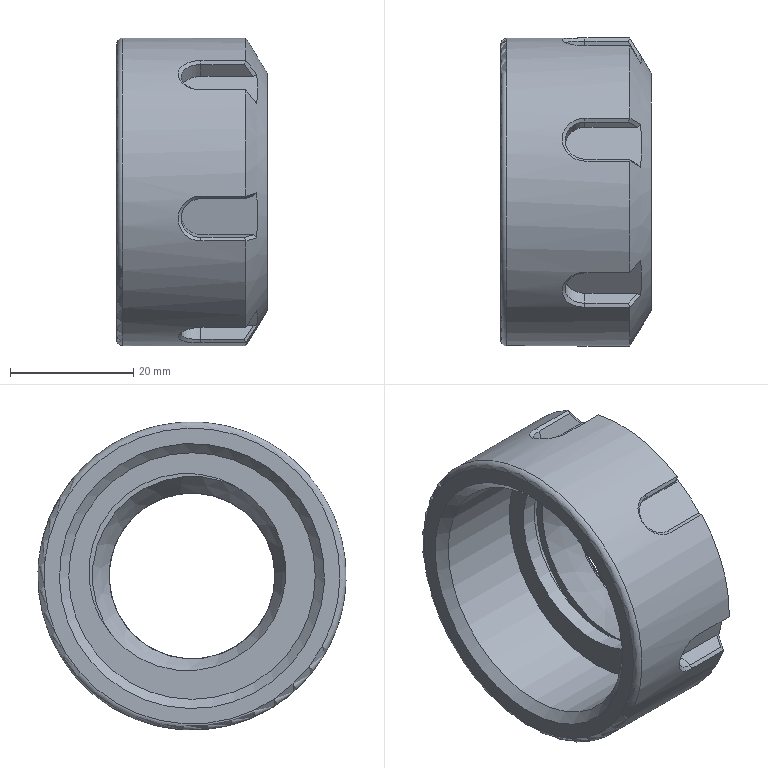Component | NX | 12_02_NUT_ER32UM | 1 solid | 77 faces | volume 18866 mm3 | plane 42 | spline 18 | cylinder 11 | cone 3 | torus 3 | commonest cylinder face diameters 6.4 x6 40 x1 32 x1 35 x1 26.9 x1 50 x1